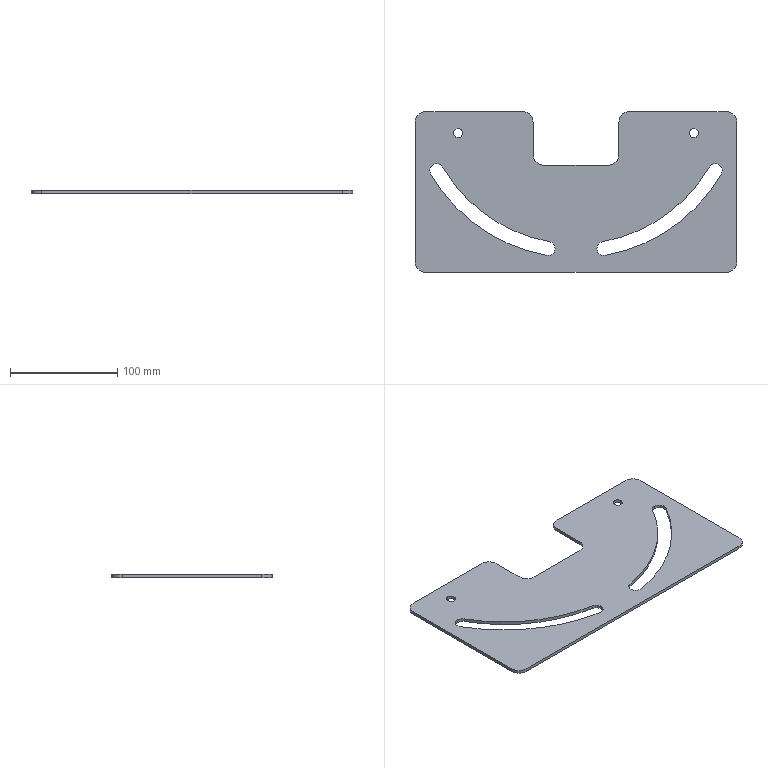Component | SolidWorks | KSD171005A-01-01-32-1 | 1 solid | 32 faces | box 300 x 150 x 3 mm | volume 111395 mm3 | cylinder 22 | plane 10 | commonest cylinder face diameters 20 x8 13 x6 8.5 x4 287 x2 313 x2
build123d program:
from build123d import *

# Parameters (mm, degrees)
SKETCH1_W                      = 150
SKETCH1_H                      = 300
BOSS_EXTRUDE1_DEPTH            = 3
CUT_EXTRUDE2_DEPTH             = 10
FILLET1_R                      = 10
SKETCH5_W                      = 100
SKETCH5_H                      = 80
CUT_EXTRUDE3_DEPTH             = 10
F_8_5_8_5_DIAMETER_HOLE1_D     = 8.5
F_8_5_8_5_DIAMETER_HOLE1_DEPTH = 11
F_8_5_8_5_DIAMETER_HOLE1_TIP   = 2.554
FILLET2_R                      = 10


with BuildPart() as part:
    # Sketch1 → Boss-Extrude1 (new body)
    with BuildSketch(Plane.XY):
        Rectangle(SKETCH1_W, SKETCH1_H)
    extrude(amount=BOSS_EXTRUDE1_DEPTH)

    # Sketch4 → Cut-Extrude2 (cut)
    with BuildSketch(Plane.XY.offset(3)):
        with BuildLine():
            ThreePointArc((16.75, 135.533), (-33.197, 89.765), (-59.122, 27.176))
            ThreePointArc((-59.122, 27.176), (-53.85, 19.646), (-46.32, 24.919))
            ThreePointArc((-46.32, 24.919), (-22.548, 82.308), (23.25, 124.275))
            ThreePointArc((23.25, 124.275), (25.629, 133.154), (16.75, 135.533))
        make_face()
        with BuildLine():
            ThreePointArc((16.75, -135.533), (-33.197, -89.765), (-59.122, -27.176))
            ThreePointArc((-59.122, -27.176), (-53.85, -19.646), (-46.32, -24.919))
            ThreePointArc((-46.32, -24.919), (-22.548, -82.308), (23.25, -124.275))
            ThreePointArc((23.25, -124.275), (25.629, -133.154), (16.75, -135.533))
        make_face()
    extrude(amount=-CUT_EXTRUDE2_DEPTH, mode=Mode.SUBTRACT)

    # Fillet1
    fillet1_edges = [part.edges().sort_by_distance(p)[0] for p in [
        (75, -150, 1.5),
        (-75, -150, 1.5),
        (-75, 150, 1.5),
        (75, 150, 1.5),
    ]]
    fillet(fillet1_edges, radius=FILLET1_R)

    # Sketch5 → Cut-Extrude3 (cut)
    with BuildSketch(Plane.XY.offset(3)):
        with Locations((75, 0)):
            Rectangle(SKETCH5_W, SKETCH5_H)
    extrude(amount=-CUT_EXTRUDE3_DEPTH, mode=Mode.SUBTRACT)

    # 8.5 _8.5_ Diameter Hole1
    with Locations(Plane.XY.offset(3)):
        with Locations((55, 110), (55, -110)):
            Hole(F_8_5_8_5_DIAMETER_HOLE1_D / 2, depth=F_8_5_8_5_DIAMETER_HOLE1_DEPTH)
            with Locations((0, 0, -(F_8_5_8_5_DIAMETER_HOLE1_DEPTH + F_8_5_8_5_DIAMETER_HOLE1_TIP / 2))):  # 118° drill point
                Cone(0, F_8_5_8_5_DIAMETER_HOLE1_D / 2, F_8_5_8_5_DIAMETER_HOLE1_TIP, mode=Mode.SUBTRACT)

    # Fillet2
    fillet2_edges = [part.edges().sort_by_distance(p)[0] for p in [
        (75, 40, 1.5),
        (75, -40, 1.5),
        (25, -40, 1.5),
        (25, 40, 1.5),
    ]]
    fillet(fillet2_edges, radius=FILLET2_R)


solid = part.part

# Placed as in the assembly
solid = solid.moved(Location((-7.111, -79.27, 348), (0, 0, 90)))
STEP:
#1=CARTESIAN_POINT('',(-4.611,-1.123,13.701));
#2=VERTEX_POINT('',#1);
#3=CARTESIAN_POINT('',(-4.611,-0.7882,13.701));
#4=VERTEX_POINT('',#3);
#5=CARTESIAN_POINT('',(-4.611,-0.9555,13.701));
#6=DIRECTION('',(-0.,-0.,1.));
#7=DIRECTION('',(0.,1.,0.));
#8=AXIS2_PLACEMENT_3D('',#5,#6,#7);
#9=CIRCLE('',#8,0.1673);
#10=EDGE_CURVE('',#2,#4,#9,.T.);
#11=ORIENTED_EDGE('',*,*,#10,.F.);
#12=CARTESIAN_POINT('',(-4.611,-1.123,13.819));
#13=VERTEX_POINT('',#12);
#14=CARTESIAN_POINT('',(-4.611,-1.123,13.819));
#15=DIRECTION('',(-0.,-0.,1.));
#16=VECTOR('',#15,39.37);
#17=LINE('',#14,#16);
#18=EDGE_CURVE('',#2,#13,#17,.T.);
#19=ORIENTED_EDGE('',*,*,#18,.T.);
#20=CARTESIAN_POINT('',(-4.611,-0.7882,13.819));
#21=VERTEX_POINT('',#20);
#22=CARTESIAN_POINT('',(-4.611,-0.9555,13.819));
#23=DIRECTION('',(-0.,-0.,1.));
#24=DIRECTION('',(0.,1.,0.));
#25=AXIS2_PLACEMENT_3D('',#22,#23,#24);
#26=CIRCLE('',#25,0.1673);
#27=EDGE_CURVE('',#13,#21,#26,.T.);
#28=ORIENTED_EDGE('',*,*,#27,.T.);
#29=CARTESIAN_POINT('',(-4.611,-0.7882,13.819));
#30=DIRECTION('',(-0.,-0.,1.));
#31=VECTOR('',#30,39.37);
#32=LINE('',#29,#31);
#33=EDGE_CURVE('',#4,#21,#32,.T.);
#34=ORIENTED_EDGE('',*,*,#33,.F.);
#35=EDGE_LOOP('',(#11,#19,#28,#34));
#36=FACE_OUTER_BOUND('',#35,.T.);
#37=CARTESIAN_POINT('',(-4.611,-0.9555,13.819));
#38=DIRECTION('',(-0.,-0.,1.));
#39=DIRECTION('',(0.,1.,0.));
#40=AXIS2_PLACEMENT_3D('',#37,#38,#39);
#41=CYLINDRICAL_SURFACE('',#40,0.1673);
#42=ADVANCED_FACE('',(#36),#41,.F.);
#43=CARTESIAN_POINT('',(4.051,-1.123,13.701));
#44=VERTEX_POINT('',#43);
#45=CARTESIAN_POINT('',(4.051,-0.7882,13.701));
#46=VERTEX_POINT('',#45);
#47=CARTESIAN_POINT('',(4.051,-0.9555,13.701));
#48=DIRECTION('',(-0.,-0.,1.));
#49=DIRECTION('',(0.,1.,0.));
#50=AXIS2_PLACEMENT_3D('',#47,#48,#49);
#51=CIRCLE('',#50,0.1673);
#52=EDGE_CURVE('',#44,#46,#51,.T.);
#53=ORIENTED_EDGE('',*,*,#52,.F.);
#54=CARTESIAN_POINT('',(4.051,-1.123,13.819));
#55=VERTEX_POINT('',#54);
#56=CARTESIAN_POINT('',(4.051,-1.123,13.819));
#57=DIRECTION('',(-0.,-0.,1.));
#58=VECTOR('',#57,39.37);
#59=LINE('',#56,#58);
#60=EDGE_CURVE('',#44,#55,#59,.T.);
#61=ORIENTED_EDGE('',*,*,#60,.T.);
#62=CARTESIAN_POINT('',(4.051,-0.7882,13.819));
#63=VERTEX_POINT('',#62);
#64=CARTESIAN_POINT('',(4.051,-0.9555,13.819));
#65=DIRECTION('',(-0.,-0.,1.));
#66=DIRECTION('',(0.,1.,0.));
#67=AXIS2_PLACEMENT_3D('',#64,#65,#66);
#68=CIRCLE('',#67,0.1673);
#69=EDGE_CURVE('',#55,#63,#68,.T.);
#70=ORIENTED_EDGE('',*,*,#69,.T.);
#71=CARTESIAN_POINT('',(4.051,-0.7882,13.819));
#72=DIRECTION('',(-0.,-0.,1.));
#73=VECTOR('',#72,39.37);
#74=LINE('',#71,#73);
#75=EDGE_CURVE('',#46,#63,#74,.T.);
#76=ORIENTED_EDGE('',*,*,#75,.F.);
#77=EDGE_LOOP('',(#53,#61,#70,#76));
#78=FACE_OUTER_BOUND('',#77,.T.);
#79=CARTESIAN_POINT('',(4.051,-0.9555,13.819));
#80=DIRECTION('',(-0.,-0.,1.));
#81=DIRECTION('',(0.,1.,0.));
#82=AXIS2_PLACEMENT_3D('',#79,#80,#81);
#83=CYLINDRICAL_SURFACE('',#82,0.1673);
#84=ADVANCED_FACE('',(#78),#83,.F.);
#85=CARTESIAN_POINT('',(4.834,-2.078,13.701));
#86=VERTEX_POINT('',#85);
#87=CARTESIAN_POINT('',(4.613,-2.206,13.701));
#88=VERTEX_POINT('',#87);
#89=CARTESIAN_POINT('',(4.834,-2.333,13.701));
#90=DIRECTION('',(-0.,-0.,1.));
#91=DIRECTION('',(0.,1.,0.));
#92=AXIS2_PLACEMENT_3D('',#89,#90,#91);
#93=CIRCLE('',#92,0.2559);
#94=EDGE_CURVE('',#86,#88,#93,.T.);
#95=ORIENTED_EDGE('',*,*,#94,.F.);
#96=CARTESIAN_POINT('',(4.834,-2.078,13.819));
#97=VERTEX_POINT('',#96);
#98=CARTESIAN_POINT('',(4.834,-2.078,13.425));
#99=DIRECTION('',(-0.,-0.,1.));
#100=VECTOR('',#99,39.37);
#101=LINE('',#98,#100);
#102=EDGE_CURVE('',#86,#97,#101,.T.);
#103=ORIENTED_EDGE('',*,*,#102,.T.);
#104=CARTESIAN_POINT('',(4.613,-2.206,13.819));
#105=VERTEX_POINT('',#104);
#106=CARTESIAN_POINT('',(4.834,-2.333,13.819));
#107=DIRECTION('',(-0.,-0.,1.));
#108=DIRECTION('',(0.,-1.,0.));
#109=AXIS2_PLACEMENT_3D('',#106,#107,#108);
#110=CIRCLE('',#109,0.2559);
#111=EDGE_CURVE('',#97,#105,#110,.T.);
#112=ORIENTED_EDGE('',*,*,#111,.T.);
#113=CARTESIAN_POINT('',(4.613,-2.206,13.425));
#114=DIRECTION('',(-0.,-0.,1.));
#115=VECTOR('',#114,39.37);
#116=LINE('',#113,#115);
#117=EDGE_CURVE('',#88,#105,#116,.T.);
#118=ORIENTED_EDGE('',*,*,#117,.F.);
#119=EDGE_LOOP('',(#95,#103,#112,#118));
#120=FACE_OUTER_BOUND('',#119,.T.);
#121=CARTESIAN_POINT('',(4.834,-2.333,13.425));
#122=DIRECTION('',(-0.,-0.,1.));
#123=DIRECTION('',(0.,1.,0.));
#124=AXIS2_PLACEMENT_3D('',#121,#122,#123);
#125=CYLINDRICAL_SURFACE('',#124,0.2559);
#126=ADVANCED_FACE('',(#120),#125,.F.);
#127=CARTESIAN_POINT('',(-5.394,-2.078,13.701));
#128=VERTEX_POINT('',#127);
#129=CARTESIAN_POINT('',(-5.616,-2.461,13.701));
#130=VERTEX_POINT('',#129);
#131=CARTESIAN_POINT('',(-5.394,-2.333,13.701));
#132=DIRECTION('',(-0.,-0.,1.));
#133=DIRECTION('',(0.,1.,0.));
#134=AXIS2_PLACEMENT_3D('',#131,#132,#133);
#135=CIRCLE('',#134,0.2559);
#136=EDGE_CURVE('',#128,#130,#135,.T.);
#137=ORIENTED_EDGE('',*,*,#136,.F.);
#138=CARTESIAN_POINT('',(-5.394,-2.078,13.819));
#139=VERTEX_POINT('',#138);
#140=CARTESIAN_POINT('',(-5.394,-2.078,13.425));
#141=DIRECTION('',(-0.,-0.,1.));
#142=VECTOR('',#141,39.37);
#143=LINE('',#140,#142);
#144=EDGE_CURVE('',#128,#139,#143,.T.);
#145=ORIENTED_EDGE('',*,*,#144,.T.);
#146=CARTESIAN_POINT('',(-5.616,-2.461,13.819));
#147=VERTEX_POINT('',#146);
#148=CARTESIAN_POINT('',(-5.394,-2.333,13.819));
#149=DIRECTION('',(-0.,-0.,1.));
#150=DIRECTION('',(0.,1.,0.));
#151=AXIS2_PLACEMENT_3D('',#148,#149,#150);
#152=CIRCLE('',#151,0.2559);
#153=EDGE_CURVE('',#139,#147,#152,.T.);
#154=ORIENTED_EDGE('',*,*,#153,.T.);
#155=CARTESIAN_POINT('',(-5.616,-2.461,13.425));
#156=DIRECTION('',(-0.,-0.,1.));
#157=VECTOR('',#156,39.37);
#158=LINE('',#155,#157);
#159=EDGE_CURVE('',#130,#147,#158,.T.);
#160=ORIENTED_EDGE('',*,*,#159,.F.);
#161=EDGE_LOOP('',(#137,#145,#154,#160));
#162=FACE_OUTER_BOUND('',#161,.T.);
#163=CARTESIAN_POINT('',(-5.394,-2.333,13.425));
#164=DIRECTION('',(-0.,-0.,1.));
#165=DIRECTION('',(0.,1.,0.));
#166=AXIS2_PLACEMENT_3D('',#163,#164,#165);
#167=CYLINDRICAL_SURFACE('',#166,0.2559);
#168=ADVANCED_FACE('',(#162),#167,.F.);
#169=CARTESIAN_POINT('',(5.232,-0.1681,13.701));
#170=VERTEX_POINT('',#169);
#171=CARTESIAN_POINT('',(1.689,-0.1681,13.701));
#172=VERTEX_POINT('',#171);
#173=CARTESIAN_POINT('',(-6.185,-0.1681,13.701));
#174=DIRECTION('',(-1.,0.,-0.));
#175=VECTOR('',#174,39.37);
#176=LINE('',#173,#175);
#177=EDGE_CURVE('',#170,#172,#176,.T.);
#178=ORIENTED_EDGE('',*,*,#177,.T.);
#179=CARTESIAN_POINT('',(1.689,-0.1681,13.819));
#180=VERTEX_POINT('',#179);
#181=CARTESIAN_POINT('',(1.689,-0.1681,13.819));
#182=DIRECTION('',(-0.,-0.,1.));
#183=VECTOR('',#182,39.37);
#184=LINE('',#181,#183);
#185=EDGE_CURVE('',#172,#180,#184,.T.);
#186=ORIENTED_EDGE('',*,*,#185,.T.);
#187=CARTESIAN_POINT('',(5.232,-0.1681,13.819));
#188=VERTEX_POINT('',#187);
#189=CARTESIAN_POINT('',(-6.185,-0.1681,13.819));
#190=DIRECTION('',(-1.,0.,-0.));
#191=VECTOR('',#190,39.37);
#192=LINE('',#189,#191);
#193=EDGE_CURVE('',#188,#180,#192,.T.);
#194=ORIENTED_EDGE('',*,*,#193,.F.);
#195=CARTESIAN_POINT('',(5.232,-0.1681,13.819));
#196=DIRECTION('',(0.,0.,-1.));
#197=VECTOR('',#196,39.37);
#198=LINE('',#195,#197);
#199=EDGE_CURVE('',#188,#170,#198,.T.);
#200=ORIENTED_EDGE('',*,*,#199,.T.);
#201=EDGE_LOOP('',(#178,#186,#194,#200));
#202=FACE_OUTER_BOUND('',#201,.T.);
#203=CARTESIAN_POINT('',(-6.185,-0.1681,13.819));
#204=DIRECTION('',(-0.,-1.,-0.));
#205=DIRECTION('',(1.,-0.,0.));
#206=AXIS2_PLACEMENT_3D('',#203,#204,#205);
#207=PLANE('',#206);
#208=ADVANCED_FACE('',(#202),#207,.F.);
#209=CARTESIAN_POINT('',(-4.611,-0.9555,13.819));
#210=DIRECTION('',(-0.,-0.,1.));
#211=DIRECTION('',(0.,1.,0.));
#212=AXIS2_PLACEMENT_3D('',#209,#210,#211);
#213=CIRCLE('',#212,0.1673);
#214=EDGE_CURVE('',#21,#13,#213,.T.);
#215=ORIENTED_EDGE('',*,*,#214,.F.);
#216=ORIENTED_EDGE('',*,*,#27,.F.);
#217=EDGE_LOOP('',(#215,#216));
#218=FACE_BOUND('',#217,.T.);
#219=CARTESIAN_POINT('',(4.051,-0.9555,13.819));
#220=DIRECTION('',(-0.,-0.,1.));
#221=DIRECTION('',(0.,1.,0.));
#222=AXIS2_PLACEMENT_3D('',#219,#220,#221);
#223=CIRCLE('',#222,0.1673);
#224=EDGE_CURVE('',#63,#55,#223,.T.);
#225=ORIENTED_EDGE('',*,*,#224,.F.);
#226=ORIENTED_EDGE('',*,*,#69,.F.);
#227=EDGE_LOOP('',(#225,#226));
#228=FACE_BOUND('',#227,.T.);
#229=ORIENTED_EDGE('',*,*,#193,.T.);
#230=CARTESIAN_POINT('',(1.295,-0.5618,13.819));
#231=VERTEX_POINT('',#230);
#232=CARTESIAN_POINT('',(1.689,-0.5618,13.819));
#233=DIRECTION('',(-0.,-0.,1.));
#234=DIRECTION('',(0.,1.,0.));
#235=AXIS2_PLACEMENT_3D('',#232,#233,#234);
#236=CIRCLE('',#235,0.3937);
#237=EDGE_CURVE('',#180,#231,#236,.T.);
#238=ORIENTED_EDGE('',*,*,#237,.T.);
#239=CARTESIAN_POINT('',(1.295,-1.743,13.819));
#240=VERTEX_POINT('',#239);
#241=CARTESIAN_POINT('',(1.295,-2.137,13.819));
#242=DIRECTION('',(0.,1.,0.));
#243=VECTOR('',#242,39.37);
#244=LINE('',#241,#243);
#245=EDGE_CURVE('',#240,#231,#244,.T.);
#246=ORIENTED_EDGE('',*,*,#245,.F.);
#247=CARTESIAN_POINT('',(0.9011,-2.137,13.819));
#248=VERTEX_POINT('',#247);
#249=CARTESIAN_POINT('',(0.9011,-1.743,13.819));
#250=DIRECTION('',(0.,0.,-1.));
#251=DIRECTION('',(0.,1.,0.));
#252=AXIS2_PLACEMENT_3D('',#249,#250,#251);
#253=CIRCLE('',#252,0.3937);
#254=EDGE_CURVE('',#240,#248,#253,.T.);
#255=ORIENTED_EDGE('',*,*,#254,.T.);
#256=CARTESIAN_POINT('',(-1.461,-2.137,13.819));
#257=VERTEX_POINT('',#256);
#258=CARTESIAN_POINT('',(-1.855,-2.137,13.819));
#259=DIRECTION('',(1.,-0.,0.));
#260=VECTOR('',#259,39.37);
#261=LINE('',#258,#260);
#262=EDGE_CURVE('',#257,#248,#261,.T.);
#263=ORIENTED_EDGE('',*,*,#262,.F.);
#264=CARTESIAN_POINT('',(-1.855,-1.743,13.819));
#265=VERTEX_POINT('',#264);
#266=CARTESIAN_POINT('',(-1.461,-1.743,13.819));
#267=DIRECTION('',(0.,0.,-1.));
#268=DIRECTION('',(0.,1.,0.));
#269=AXIS2_PLACEMENT_3D('',#266,#267,#268);
#270=CIRCLE('',#269,0.3937);
#271=EDGE_CURVE('',#257,#265,#270,.T.);
#272=ORIENTED_EDGE('',*,*,#271,.T.);
#273=CARTESIAN_POINT('',(-1.855,-0.5618,13.819));
#274=VERTEX_POINT('',#273);
#275=CARTESIAN_POINT('',(-1.855,-2.137,13.819));
#276=DIRECTION('',(-0.,-1.,-0.));
#277=VECTOR('',#276,39.37);
#278=LINE('',#275,#277);
#279=EDGE_CURVE('',#274,#265,#278,.T.);
#280=ORIENTED_EDGE('',*,*,#279,.F.);
#281=CARTESIAN_POINT('',(-2.248,-0.1681,13.819));
#282=VERTEX_POINT('',#281);
#283=CARTESIAN_POINT('',(-2.248,-0.5618,13.819));
#284=DIRECTION('',(-0.,-0.,1.));
#285=DIRECTION('',(0.,1.,0.));
#286=AXIS2_PLACEMENT_3D('',#283,#284,#285);
#287=CIRCLE('',#286,0.3937);
#288=EDGE_CURVE('',#274,#282,#287,.T.);
#289=ORIENTED_EDGE('',*,*,#288,.T.);
#290=CARTESIAN_POINT('',(-5.792,-0.1681,13.819));
#291=VERTEX_POINT('',#290);
#292=CARTESIAN_POINT('',(-6.185,-0.1681,13.819));
#293=DIRECTION('',(-1.,0.,-0.));
#294=VECTOR('',#293,39.37);
#295=LINE('',#292,#294);
#296=EDGE_CURVE('',#282,#291,#295,.T.);
#297=ORIENTED_EDGE('',*,*,#296,.T.);
#298=CARTESIAN_POINT('',(-6.185,-0.5618,13.819));
#299=VERTEX_POINT('',#298);
#300=CARTESIAN_POINT('',(-5.792,-0.5618,13.819));
#301=DIRECTION('',(-0.,-0.,1.));
#302=DIRECTION('',(0.,1.,0.));
#303=AXIS2_PLACEMENT_3D('',#300,#301,#302);
#304=CIRCLE('',#303,0.3937);
#305=EDGE_CURVE('',#291,#299,#304,.T.);
#306=ORIENTED_EDGE('',*,*,#305,.T.);
#307=CARTESIAN_POINT('',(-6.185,-5.68,13.819));
#308=VERTEX_POINT('',#307);
#309=CARTESIAN_POINT('',(-6.185,-6.074,13.819));
#310=DIRECTION('',(-0.,-1.,-0.));
#311=VECTOR('',#310,39.37);
#312=LINE('',#309,#311);
#313=EDGE_CURVE('',#299,#308,#312,.T.);
#314=ORIENTED_EDGE('',*,*,#313,.T.);
#315=CARTESIAN_POINT('',(-5.792,-6.074,13.819));
#316=VERTEX_POINT('',#315);
#317=CARTESIAN_POINT('',(-5.792,-5.68,13.819));
#318=DIRECTION('',(-0.,-0.,1.));
#319=DIRECTION('',(0.,1.,0.));
#320=AXIS2_PLACEMENT_3D('',#317,#318,#319);
#321=CIRCLE('',#320,0.3937);
#322=EDGE_CURVE('',#308,#316,#321,.T.);
#323=ORIENTED_EDGE('',*,*,#322,.T.);
#324=CARTESIAN_POINT('',(5.232,-6.074,13.819));
#325=VERTEX_POINT('',#324);
#326=CARTESIAN_POINT('',(-6.185,-6.074,13.819));
#327=DIRECTION('',(1.,-0.,0.));
#328=VECTOR('',#327,39.37);
#329=LINE('',#326,#328);
#330=EDGE_CURVE('',#316,#325,#329,.T.);
#331=ORIENTED_EDGE('',*,*,#330,.T.);
#332=CARTESIAN_POINT('',(5.626,-5.68,13.819));
#333=VERTEX_POINT('',#332);
#334=CARTESIAN_POINT('',(5.232,-5.68,13.819));
#335=DIRECTION('',(-0.,-0.,1.));
#336=DIRECTION('',(0.,1.,0.));
#337=AXIS2_PLACEMENT_3D('',#334,#335,#336);
#338=CIRCLE('',#337,0.3937);
#339=EDGE_CURVE('',#325,#333,#338,.T.);
#340=ORIENTED_EDGE('',*,*,#339,.T.);
#341=CARTESIAN_POINT('',(5.626,-0.5618,13.819));
#342=VERTEX_POINT('',#341);
#343=CARTESIAN_POINT('',(5.626,-6.074,13.819));
#344=DIRECTION('',(0.,1.,0.));
#345=VECTOR('',#344,39.37);
#346=LINE('',#343,#345);
#347=EDGE_CURVE('',#333,#342,#346,.T.);
#348=ORIENTED_EDGE('',*,*,#347,.T.);
#349=CARTESIAN_POINT('',(5.232,-0.5618,13.819));
#350=DIRECTION('',(-0.,-0.,1.));
#351=DIRECTION('',(0.,1.,0.));
#352=AXIS2_PLACEMENT_3D('',#349,#350,#351);
#353=CIRCLE('',#352,0.3937);
#354=EDGE_CURVE('',#342,#188,#353,.T.);
#355=ORIENTED_EDGE('',*,*,#354,.T.);
#356=EDGE_LOOP('',(#229,#238,#246,#255,#263,#272,#280,#289,#297,#306,#314,#323,#331,#340,#348,#355));
#357=FACE_OUTER_BOUND('',#356,.T.);
#358=CARTESIAN_POINT('',(-5.173,-2.206,13.819));
#359=VERTEX_POINT('',#358);
#360=CARTESIAN_POINT('',(-5.394,-2.333,13.819));
#361=DIRECTION('',(-0.,-0.,1.));
#362=DIRECTION('',(0.,1.,0.));
#363=AXIS2_PLACEMENT_3D('',#360,#361,#362);
#364=CIRCLE('',#363,0.2559);
#365=EDGE_CURVE('',#359,#139,#364,.T.);
#366=ORIENTED_EDGE('',*,*,#365,.F.);
#367=CARTESIAN_POINT('',(-1.261,-4.944,13.819));
#368=VERTEX_POINT('',#367);
#369=CARTESIAN_POINT('',(-0.28,0.6193,13.819));
#370=DIRECTION('',(0.,0.,-1.));
#371=DIRECTION('',(0.,1.,0.));
#372=AXIS2_PLACEMENT_3D('',#369,#370,#371);
#373=CIRCLE('',#372,5.65);
#374=EDGE_CURVE('',#368,#359,#373,.T.);
#375=ORIENTED_EDGE('',*,*,#374,.F.);
#376=CARTESIAN_POINT('',(-1.35,-5.449,13.819));
#377=VERTEX_POINT('',#376);
#378=CARTESIAN_POINT('',(-1.305,-5.197,13.819));
#379=DIRECTION('',(-0.,-0.,1.));
#380=DIRECTION('',(0.,1.,0.));
#381=AXIS2_PLACEMENT_3D('',#378,#379,#380);
#382=CIRCLE('',#381,0.2559);
#383=EDGE_CURVE('',#377,#368,#382,.T.);
#384=ORIENTED_EDGE('',*,*,#383,.F.);
#385=CARTESIAN_POINT('',(-0.28,0.6193,13.819));
#386=DIRECTION('',(-0.,-0.,1.));
#387=DIRECTION('',(0.,1.,0.));
#388=AXIS2_PLACEMENT_3D('',#385,#386,#387);
#389=CIRCLE('',#388,6.161);
#390=EDGE_CURVE('',#147,#377,#389,.T.);
#391=ORIENTED_EDGE('',*,*,#390,.F.);
#392=ORIENTED_EDGE('',*,*,#153,.F.);
#393=EDGE_LOOP('',(#366,#375,#384,#391,#392));
#394=FACE_BOUND('',#393,.T.);
#395=CARTESIAN_POINT('',(5.056,-2.461,13.819));
#396=VERTEX_POINT('',#395);
#397=CARTESIAN_POINT('',(4.834,-2.333,13.819));
#398=DIRECTION('',(-0.,-0.,1.));
#399=DIRECTION('',(0.,-1.,0.));
#400=AXIS2_PLACEMENT_3D('',#397,#398,#399);
#401=CIRCLE('',#400,0.2559);
#402=EDGE_CURVE('',#396,#97,#401,.T.);
#403=ORIENTED_EDGE('',*,*,#402,.F.);
#404=CARTESIAN_POINT('',(0.7899,-5.449,13.819));
#405=VERTEX_POINT('',#404);
#406=CARTESIAN_POINT('',(-0.28,0.6193,13.819));
#407=DIRECTION('',(-0.,-0.,1.));
#408=DIRECTION('',(-0.,-1.,0.));
#409=AXIS2_PLACEMENT_3D('',#406,#407,#408);
#410=CIRCLE('',#409,6.161);
#411=EDGE_CURVE('',#405,#396,#410,.T.);
#412=ORIENTED_EDGE('',*,*,#411,.F.);
#413=CARTESIAN_POINT('',(0.7011,-4.944,13.819));
#414=VERTEX_POINT('',#413);
#415=CARTESIAN_POINT('',(0.7455,-5.197,13.819));
#416=DIRECTION('',(-0.,-0.,1.));
#417=DIRECTION('',(0.,-1.,0.));
#418=AXIS2_PLACEMENT_3D('',#415,#416,#417);
#419=CIRCLE('',#418,0.2559);
#420=EDGE_CURVE('',#414,#405,#419,.T.);
#421=ORIENTED_EDGE('',*,*,#420,.F.);
#422=CARTESIAN_POINT('',(-0.28,0.6193,13.819));
#423=DIRECTION('',(0.,0.,-1.));
#424=DIRECTION('',(-0.,-1.,0.));
#425=AXIS2_PLACEMENT_3D('',#422,#423,#424);
#426=CIRCLE('',#425,5.65);
#427=EDGE_CURVE('',#105,#414,#426,.T.);
#428=ORIENTED_EDGE('',*,*,#427,.F.);
#429=ORIENTED_EDGE('',*,*,#111,.F.);
#430=EDGE_LOOP('',(#403,#412,#421,#428,#429));
#431=FACE_BOUND('',#430,.T.);
#432=CARTESIAN_POINT('',(-0.28,-3.121,13.819));
#433=DIRECTION('',(-0.,-0.,1.));
#434=DIRECTION('',(0.,1.,0.));
#435=AXIS2_PLACEMENT_3D('',#432,#433,#434);
#436=PLANE('',#435);
#437=ADVANCED_FACE('',(#218,#228,#357,#394,#431),#436,.T.);
#438=CARTESIAN_POINT('',(-4.611,-0.9555,13.701));
#439=DIRECTION('',(-0.,-0.,1.));
#440=DIRECTION('',(0.,1.,0.));
#441=AXIS2_PLACEMENT_3D('',#438,#439,#440);
#442=CIRCLE('',#441,0.1673);
#443=EDGE_CURVE('',#4,#2,#442,.T.);
#444=ORIENTED_EDGE('',*,*,#443,.T.);
#445=ORIENTED_EDGE('',*,*,#10,.T.);
#446=EDGE_LOOP('',(#444,#445));
#447=FACE_BOUND('',#446,.T.);
#448=CARTESIAN_POINT('',(4.051,-0.9555,13.701));
#449=DIRECTION('',(-0.,-0.,1.));
#450=DIRECTION('',(0.,1.,0.));
#451=AXIS2_PLACEMENT_3D('',#448,#449,#450);
#452=CIRCLE('',#451,0.1673);
#453=EDGE_CURVE('',#46,#44,#452,.T.);
#454=ORIENTED_EDGE('',*,*,#453,.T.);
#455=ORIENTED_EDGE('',*,*,#52,.T.);
#456=EDGE_LOOP('',(#454,#455));
#457=FACE_BOUND('',#456,.T.);
#458=CARTESIAN_POINT('',(-1.261,-4.944,13.701));
#459=VERTEX_POINT('',#458);
#460=CARTESIAN_POINT('',(-5.173,-2.206,13.701));
#461=VERTEX_POINT('',#460);
#462=CARTESIAN_POINT('',(-0.28,0.6193,13.701));
#463=DIRECTION('',(0.,0.,-1.));
#464=DIRECTION('',(0.,1.,0.));
#465=AXIS2_PLACEMENT_3D('',#462,#463,#464);
#466=CIRCLE('',#465,5.65);
#467=EDGE_CURVE('',#459,#461,#466,.T.);
#468=ORIENTED_EDGE('',*,*,#467,.T.);
#469=CARTESIAN_POINT('',(-5.394,-2.333,13.701));
#470=DIRECTION('',(-0.,-0.,1.));
#471=DIRECTION('',(0.,1.,0.));
#472=AXIS2_PLACEMENT_3D('',#469,#470,#471);
#473=CIRCLE('',#472,0.2559);
#474=EDGE_CURVE('',#461,#128,#473,.T.);
#475=ORIENTED_EDGE('',*,*,#474,.T.);
#476=ORIENTED_EDGE('',*,*,#136,.T.);
#477=CARTESIAN_POINT('',(-1.35,-5.449,13.701));
#478=VERTEX_POINT('',#477);
#479=CARTESIAN_POINT('',(-0.28,0.6193,13.701));
#480=DIRECTION('',(-0.,-0.,1.));
#481=DIRECTION('',(0.,1.,0.));
#482=AXIS2_PLACEMENT_3D('',#479,#480,#481);
#483=CIRCLE('',#482,6.161);
#484=EDGE_CURVE('',#130,#478,#483,.T.);
#485=ORIENTED_EDGE('',*,*,#484,.T.);
#486=CARTESIAN_POINT('',(-1.305,-5.197,13.701));
#487=DIRECTION('',(-0.,-0.,1.));
#488=DIRECTION('',(0.,1.,0.));
#489=AXIS2_PLACEMENT_3D('',#486,#487,#488);
#490=CIRCLE('',#489,0.2559);
#491=EDGE_CURVE('',#478,#459,#490,.T.);
#492=ORIENTED_EDGE('',*,*,#491,.T.);
#493=EDGE_LOOP('',(#468,#475,#476,#485,#492));
#494=FACE_BOUND('',#493,.T.);
#495=CARTESIAN_POINT('',(1.295,-1.743,13.701));
#496=VERTEX_POINT('',#495);
#497=CARTESIAN_POINT('',(1.295,-0.5618,13.701));
#498=VERTEX_POINT('',#497);
#499=CARTESIAN_POINT('',(1.295,-3.121,13.701));
#500=DIRECTION('',(0.,1.,0.));
#501=VECTOR('',#500,39.37);
#502=LINE('',#499,#501);
#503=EDGE_CURVE('',#496,#498,#502,.T.);
#504=ORIENTED_EDGE('',*,*,#503,.T.);
#505=CARTESIAN_POINT('',(1.689,-0.5618,13.701));
#506=DIRECTION('',(0.,0.,-1.));
#507=DIRECTION('',(-0.,1.,0.));
#508=AXIS2_PLACEMENT_3D('',#505,#506,#507);
#509=CIRCLE('',#508,0.3937);
#510=EDGE_CURVE('',#498,#172,#509,.T.);
#511=ORIENTED_EDGE('',*,*,#510,.T.);
#512=ORIENTED_EDGE('',*,*,#177,.F.);
#513=CARTESIAN_POINT('',(5.626,-0.5618,13.701));
#514=VERTEX_POINT('',#513);
#515=CARTESIAN_POINT('',(5.232,-0.5618,13.701));
#516=DIRECTION('',(0.,0.,-1.));
#517=DIRECTION('',(0.,1.,0.));
#518=AXIS2_PLACEMENT_3D('',#515,#516,#517);
#519=CIRCLE('',#518,0.3937);
#520=EDGE_CURVE('',#170,#514,#519,.T.);
#521=ORIENTED_EDGE('',*,*,#520,.T.);
#522=CARTESIAN_POINT('',(5.626,-5.68,13.701));
#523=VERTEX_POINT('',#522);
#524=CARTESIAN_POINT('',(5.626,-6.074,13.701));
#525=DIRECTION('',(0.,1.,0.));
#526=VECTOR('',#525,39.37);
#527=LINE('',#524,#526);
#528=EDGE_CURVE('',#523,#514,#527,.T.);
#529=ORIENTED_EDGE('',*,*,#528,.F.);
#530=CARTESIAN_POINT('',(5.232,-6.074,13.701));
#531=VERTEX_POINT('',#530);
#532=CARTESIAN_POINT('',(5.232,-5.68,13.701));
#533=DIRECTION('',(0.,0.,-1.));
#534=DIRECTION('',(0.,1.,0.));
#535=AXIS2_PLACEMENT_3D('',#532,#533,#534);
#536=CIRCLE('',#535,0.3937);
#537=EDGE_CURVE('',#523,#531,#536,.T.);
#538=ORIENTED_EDGE('',*,*,#537,.T.);
#539=CARTESIAN_POINT('',(-5.792,-6.074,13.701));
#540=VERTEX_POINT('',#539);
#541=CARTESIAN_POINT('',(-6.185,-6.074,13.701));
#542=DIRECTION('',(1.,-0.,0.));
#543=VECTOR('',#542,39.37);
#544=LINE('',#541,#543);
#545=EDGE_CURVE('',#540,#531,#544,.T.);
#546=ORIENTED_EDGE('',*,*,#545,.F.);
#547=CARTESIAN_POINT('',(-6.185,-5.68,13.701));
#548=VERTEX_POINT('',#547);
#549=CARTESIAN_POINT('',(-5.792,-5.68,13.701));
#550=DIRECTION('',(0.,0.,-1.));
#551=DIRECTION('',(0.,1.,0.));
#552=AXIS2_PLACEMENT_3D('',#549,#550,#551);
#553=CIRCLE('',#552,0.3937);
#554=EDGE_CURVE('',#540,#548,#553,.T.);
#555=ORIENTED_EDGE('',*,*,#554,.T.);
#556=CARTESIAN_POINT('',(-6.185,-0.5618,13.701));
#557=VERTEX_POINT('',#556);
#558=CARTESIAN_POINT('',(-6.185,-6.074,13.701));
#559=DIRECTION('',(-0.,-1.,-0.));
#560=VECTOR('',#559,39.37);
#561=LINE('',#558,#560);
#562=EDGE_CURVE('',#557,#548,#561,.T.);
#563=ORIENTED_EDGE('',*,*,#562,.F.);
#564=CARTESIAN_POINT('',(-5.792,-0.1681,13.701));
#565=VERTEX_POINT('',#564);
#566=CARTESIAN_POINT('',(-5.792,-0.5618,13.701));
#567=DIRECTION('',(0.,0.,-1.));
#568=DIRECTION('',(0.,1.,0.));
#569=AXIS2_PLACEMENT_3D('',#566,#567,#568);
#570=CIRCLE('',#569,0.3937);
#571=EDGE_CURVE('',#557,#565,#570,.T.);
#572=ORIENTED_EDGE('',*,*,#571,.T.);
#573=CARTESIAN_POINT('',(-2.248,-0.1681,13.701));
#574=VERTEX_POINT('',#573);
#575=CARTESIAN_POINT('',(-6.185,-0.1681,13.701));
#576=DIRECTION('',(-1.,0.,-0.));
#577=VECTOR('',#576,39.37);
#578=LINE('',#575,#577);
#579=EDGE_CURVE('',#574,#565,#578,.T.);
#580=ORIENTED_EDGE('',*,*,#579,.F.);
#581=CARTESIAN_POINT('',(-1.855,-0.5618,13.701));
#582=VERTEX_POINT('',#581);
#583=CARTESIAN_POINT('',(-2.248,-0.5618,13.701));
#584=DIRECTION('',(0.,0.,-1.));
#585=DIRECTION('',(0.,1.,0.));
#586=AXIS2_PLACEMENT_3D('',#583,#584,#585);
#587=CIRCLE('',#586,0.3937);
#588=EDGE_CURVE('',#574,#582,#587,.T.);
#589=ORIENTED_EDGE('',*,*,#588,.T.);
#590=CARTESIAN_POINT('',(-1.855,-1.743,13.701));
#591=VERTEX_POINT('',#590);
#592=CARTESIAN_POINT('',(-1.855,-3.121,13.701));
#593=DIRECTION('',(-0.,-1.,-0.));
#594=VECTOR('',#593,39.37);
#595=LINE('',#592,#594);
#596=EDGE_CURVE('',#582,#591,#595,.T.);
#597=ORIENTED_EDGE('',*,*,#596,.T.);
#598=CARTESIAN_POINT('',(-1.461,-2.137,13.701));
#599=VERTEX_POINT('',#598);
#600=CARTESIAN_POINT('',(-1.461,-1.743,13.701));
#601=DIRECTION('',(-0.,-0.,1.));
#602=DIRECTION('',(0.,1.,0.));
#603=AXIS2_PLACEMENT_3D('',#600,#601,#602);
#604=CIRCLE('',#603,0.3937);
#605=EDGE_CURVE('',#591,#599,#604,.T.);
#606=ORIENTED_EDGE('',*,*,#605,.T.);
#607=CARTESIAN_POINT('',(0.9011,-2.137,13.701));
#608=VERTEX_POINT('',#607);
#609=CARTESIAN_POINT('',(-0.28,-2.137,13.701));
#610=DIRECTION('',(1.,-0.,0.));
#611=VECTOR('',#610,39.37);
#612=LINE('',#609,#611);
#613=EDGE_CURVE('',#599,#608,#612,.T.);
#614=ORIENTED_EDGE('',*,*,#613,.T.);
#615=CARTESIAN_POINT('',(0.9011,-1.743,13.701));
#616=DIRECTION('',(-0.,-0.,1.));
#617=DIRECTION('',(0.,1.,0.));
#618=AXIS2_PLACEMENT_3D('',#615,#616,#617);
#619=CIRCLE('',#618,0.3937);
#620=EDGE_CURVE('',#608,#496,#619,.T.);
#621=ORIENTED_EDGE('',*,*,#620,.T.);
#622=EDGE_LOOP('',(#504,#511,#512,#521,#529,#538,#546,#555,#563,#572,#580,#589,#597,#606,#614,#621));
#623=FACE_OUTER_BOUND('',#622,.T.);
#624=CARTESIAN_POINT('',(0.7899,-5.449,13.701));
#625=VERTEX_POINT('',#624);
#626=CARTESIAN_POINT('',(5.056,-2.461,13.701));
#627=VERTEX_POINT('',#626);
#628=CARTESIAN_POINT('',(-0.28,0.6193,13.701));
#629=DIRECTION('',(-0.,-0.,1.));
#630=DIRECTION('',(0.,1.,0.));
#631=AXIS2_PLACEMENT_3D('',#628,#629,#630);
#632=CIRCLE('',#631,6.161);
#633=EDGE_CURVE('',#625,#627,#632,.T.);
#634=ORIENTED_EDGE('',*,*,#633,.T.);
#635=CARTESIAN_POINT('',(4.834,-2.333,13.701));
#636=DIRECTION('',(-0.,-0.,1.));
#637=DIRECTION('',(0.,1.,0.));
#638=AXIS2_PLACEMENT_3D('',#635,#636,#637);
#639=CIRCLE('',#638,0.2559);
#640=EDGE_CURVE('',#627,#86,#639,.T.);
#641=ORIENTED_EDGE('',*,*,#640,.T.);
#642=ORIENTED_EDGE('',*,*,#94,.T.);
#643=CARTESIAN_POINT('',(0.7011,-4.944,13.701));
#644=VERTEX_POINT('',#643);
#645=CARTESIAN_POINT('',(-0.28,0.6193,13.701));
#646=DIRECTION('',(0.,0.,-1.));
#647=DIRECTION('',(0.,1.,0.));
#648=AXIS2_PLACEMENT_3D('',#645,#646,#647);
#649=CIRCLE('',#648,5.65);
#650=EDGE_CURVE('',#88,#644,#649,.T.);
#651=ORIENTED_EDGE('',*,*,#650,.T.);
#652=CARTESIAN_POINT('',(0.7455,-5.197,13.701));
#653=DIRECTION('',(-0.,-0.,1.));
#654=DIRECTION('',(0.,1.,0.));
#655=AXIS2_PLACEMENT_3D('',#652,#653,#654);
#656=CIRCLE('',#655,0.2559);
#657=EDGE_CURVE('',#644,#625,#656,.T.);
#658=ORIENTED_EDGE('',*,*,#657,.T.);
#659=EDGE_LOOP('',(#634,#641,#642,#651,#658));
#660=FACE_BOUND('',#659,.T.);
#661=CARTESIAN_POINT('',(-0.28,-3.121,13.701));
#662=DIRECTION('',(-0.,-0.,1.));
#663=DIRECTION('',(0.,1.,0.));
#664=AXIS2_PLACEMENT_3D('',#661,#662,#663);
#665=PLANE('',#664);
#666=ADVANCED_FACE('',(#447,#457,#494,#623,#660),#665,.F.);
#667=ORIENTED_EDGE('',*,*,#296,.F.);
#668=CARTESIAN_POINT('',(-2.248,-0.1681,13.819));
#669=DIRECTION('',(0.,0.,-1.));
#670=VECTOR('',#669,39.37);
#671=LINE('',#668,#670);
#672=EDGE_CURVE('',#282,#574,#671,.T.);
#673=ORIENTED_EDGE('',*,*,#672,.T.);
#674=ORIENTED_EDGE('',*,*,#579,.T.);
#675=CARTESIAN_POINT('',(-5.792,-0.1681,13.819));
#676=DIRECTION('',(-0.,-0.,1.));
#677=VECTOR('',#676,39.37);
#678=LINE('',#675,#677);
#679=EDGE_CURVE('',#565,#291,#678,.T.);
#680=ORIENTED_EDGE('',*,*,#679,.T.);
#681=EDGE_LOOP('',(#667,#673,#674,#680));
#682=FACE_OUTER_BOUND('',#681,.T.);
#683=CARTESIAN_POINT('',(-6.185,-0.1681,13.819));
#684=DIRECTION('',(-0.,-1.,-0.));
#685=DIRECTION('',(1.,-0.,0.));
#686=AXIS2_PLACEMENT_3D('',#683,#684,#685);
#687=PLANE('',#686);
#688=ADVANCED_FACE('',(#682),#687,.F.);
#689=ORIENTED_EDGE('',*,*,#313,.F.);
#690=CARTESIAN_POINT('',(-6.185,-0.5618,13.819));
#691=DIRECTION('',(0.,0.,-1.));
#692=VECTOR('',#691,39.37);
#693=LINE('',#690,#692);
#694=EDGE_CURVE('',#299,#557,#693,.T.);
#695=ORIENTED_EDGE('',*,*,#694,.T.);
#696=ORIENTED_EDGE('',*,*,#562,.T.);
#697=CARTESIAN_POINT('',(-6.185,-5.68,13.819));
#698=DIRECTION('',(-0.,-0.,1.));
#699=VECTOR('',#698,39.37);
#700=LINE('',#697,#699);
#701=EDGE_CURVE('',#548,#308,#700,.T.);
#702=ORIENTED_EDGE('',*,*,#701,.T.);
#703=EDGE_LOOP('',(#689,#695,#696,#702));
#704=FACE_OUTER_BOUND('',#703,.T.);
#705=CARTESIAN_POINT('',(-6.185,-6.074,13.819));
#706=DIRECTION('',(1.,-0.,0.));
#707=DIRECTION('',(0.,0.,-1.));
#708=AXIS2_PLACEMENT_3D('',#705,#706,#707);
#709=PLANE('',#708);
#710=ADVANCED_FACE('',(#704),#709,.F.);
#711=ORIENTED_EDGE('',*,*,#545,.T.);
#712=CARTESIAN_POINT('',(5.232,-6.074,13.819));
#713=DIRECTION('',(-0.,-0.,1.));
#714=VECTOR('',#713,39.37);
#715=LINE('',#712,#714);
#716=EDGE_CURVE('',#531,#325,#715,.T.);
#717=ORIENTED_EDGE('',*,*,#716,.T.);
#718=ORIENTED_EDGE('',*,*,#330,.F.);
#719=CARTESIAN_POINT('',(-5.792,-6.074,13.819));
#720=DIRECTION('',(0.,0.,-1.));
#721=VECTOR('',#720,39.37);
#722=LINE('',#719,#721);
#723=EDGE_CURVE('',#316,#540,#722,.T.);
#724=ORIENTED_EDGE('',*,*,#723,.T.);
#725=EDGE_LOOP('',(#711,#717,#718,#724));
#726=FACE_OUTER_BOUND('',#725,.T.);
#727=CARTESIAN_POINT('',(-6.185,-6.074,13.819));
#728=DIRECTION('',(0.,1.,0.));
#729=DIRECTION('',(-1.,0.,-0.));
#730=AXIS2_PLACEMENT_3D('',#727,#728,#729);
#731=PLANE('',#730);
#732=ADVANCED_FACE('',(#726),#731,.F.);
#733=ORIENTED_EDGE('',*,*,#347,.F.);
#734=CARTESIAN_POINT('',(5.626,-5.68,13.819));
#735=DIRECTION('',(0.,0.,-1.));
#736=VECTOR('',#735,39.37);
#737=LINE('',#734,#736);
#738=EDGE_CURVE('',#333,#523,#737,.T.);
#739=ORIENTED_EDGE('',*,*,#738,.T.);
#740=ORIENTED_EDGE('',*,*,#528,.T.);
#741=CARTESIAN_POINT('',(5.626,-0.5618,13.819));
#742=DIRECTION('',(-0.,-0.,1.));
#743=VECTOR('',#742,39.37);
#744=LINE('',#741,#743);
#745=EDGE_CURVE('',#514,#342,#744,.T.);
#746=ORIENTED_EDGE('',*,*,#745,.T.);
#747=EDGE_LOOP('',(#733,#739,#740,#746));
#748=FACE_OUTER_BOUND('',#747,.T.);
#749=CARTESIAN_POINT('',(5.626,-6.074,13.819));
#750=DIRECTION('',(-1.,0.,-0.));
#751=DIRECTION('',(-0.,-0.,1.));
#752=AXIS2_PLACEMENT_3D('',#749,#750,#751);
#753=PLANE('',#752);
#754=ADVANCED_FACE('',(#748),#753,.F.);
#755=ORIENTED_EDGE('',*,*,#144,.F.);
#756=ORIENTED_EDGE('',*,*,#474,.F.);
#757=CARTESIAN_POINT('',(-5.173,-2.206,13.425));
#758=DIRECTION('',(-0.,-0.,1.));
#759=VECTOR('',#758,39.37);
#760=LINE('',#757,#759);
#761=EDGE_CURVE('',#461,#359,#760,.T.);
#762=ORIENTED_EDGE('',*,*,#761,.T.);
#763=ORIENTED_EDGE('',*,*,#365,.T.);
#764=EDGE_LOOP('',(#755,#756,#762,#763));
#765=FACE_OUTER_BOUND('',#764,.T.);
#766=CARTESIAN_POINT('',(-5.394,-2.333,13.425));
#767=DIRECTION('',(-0.,-0.,1.));
#768=DIRECTION('',(0.,1.,0.));
#769=AXIS2_PLACEMENT_3D('',#766,#767,#768);
#770=CYLINDRICAL_SURFACE('',#769,0.2559);
#771=ADVANCED_FACE('',(#765),#770,.F.);
#772=CARTESIAN_POINT('',(-1.261,-4.944,13.425));
#773=DIRECTION('',(-0.,-0.,1.));
#774=VECTOR('',#773,39.37);
#775=LINE('',#772,#774);
#776=EDGE_CURVE('',#459,#368,#775,.T.);
#777=ORIENTED_EDGE('',*,*,#776,.T.);
#778=ORIENTED_EDGE('',*,*,#374,.T.);
#779=ORIENTED_EDGE('',*,*,#761,.F.);
#780=ORIENTED_EDGE('',*,*,#467,.F.);
#781=EDGE_LOOP('',(#777,#778,#779,#780));
#782=FACE_OUTER_BOUND('',#781,.T.);
#783=CARTESIAN_POINT('',(-0.28,0.6193,13.425));
#784=DIRECTION('',(-0.,-0.,1.));
#785=DIRECTION('',(0.,1.,0.));
#786=AXIS2_PLACEMENT_3D('',#783,#784,#785);
#787=CYLINDRICAL_SURFACE('',#786,5.65);
#788=ADVANCED_FACE('',(#782),#787,.T.);
#789=CARTESIAN_POINT('',(-1.35,-5.449,13.425));
#790=DIRECTION('',(-0.,-0.,1.));
#791=VECTOR('',#790,39.37);
#792=LINE('',#789,#791);
#793=EDGE_CURVE('',#478,#377,#792,.T.);
#794=ORIENTED_EDGE('',*,*,#793,.T.);
#795=ORIENTED_EDGE('',*,*,#383,.T.);
#796=ORIENTED_EDGE('',*,*,#776,.F.);
#797=ORIENTED_EDGE('',*,*,#491,.F.);
#798=EDGE_LOOP('',(#794,#795,#796,#797));
#799=FACE_OUTER_BOUND('',#798,.T.);
#800=CARTESIAN_POINT('',(-1.305,-5.197,13.425));
#801=DIRECTION('',(-0.,-0.,1.));
#802=DIRECTION('',(0.,1.,0.));
#803=AXIS2_PLACEMENT_3D('',#800,#801,#802);
#804=CYLINDRICAL_SURFACE('',#803,0.2559);
#805=ADVANCED_FACE('',(#799),#804,.F.);
#806=ORIENTED_EDGE('',*,*,#159,.T.);
#807=ORIENTED_EDGE('',*,*,#390,.T.);
#808=ORIENTED_EDGE('',*,*,#793,.F.);
#809=ORIENTED_EDGE('',*,*,#484,.F.);
#810=EDGE_LOOP('',(#806,#807,#808,#809));
#811=FACE_OUTER_BOUND('',#810,.T.);
#812=CARTESIAN_POINT('',(-0.28,0.6193,13.425));
#813=DIRECTION('',(-0.,-0.,1.));
#814=DIRECTION('',(0.,1.,0.));
#815=AXIS2_PLACEMENT_3D('',#812,#813,#814);
#816=CYLINDRICAL_SURFACE('',#815,6.161);
#817=ADVANCED_FACE('',(#811),#816,.F.);
#818=ORIENTED_EDGE('',*,*,#102,.F.);
#819=ORIENTED_EDGE('',*,*,#640,.F.);
#820=CARTESIAN_POINT('',(5.056,-2.461,13.425));
#821=DIRECTION('',(-0.,-0.,1.));
#822=VECTOR('',#821,39.37);
#823=LINE('',#820,#822);
#824=EDGE_CURVE('',#627,#396,#823,.T.);
#825=ORIENTED_EDGE('',*,*,#824,.T.);
#826=ORIENTED_EDGE('',*,*,#402,.T.);
#827=EDGE_LOOP('',(#818,#819,#825,#826));
#828=FACE_OUTER_BOUND('',#827,.T.);
#829=CARTESIAN_POINT('',(4.834,-2.333,13.425));
#830=DIRECTION('',(-0.,-0.,1.));
#831=DIRECTION('',(0.,1.,0.));
#832=AXIS2_PLACEMENT_3D('',#829,#830,#831);
#833=CYLINDRICAL_SURFACE('',#832,0.2559);
#834=ADVANCED_FACE('',(#828),#833,.F.);
#835=CARTESIAN_POINT('',(0.7899,-5.449,13.425));
#836=DIRECTION('',(-0.,-0.,1.));
#837=VECTOR('',#836,39.37);
#838=LINE('',#835,#837);
#839=EDGE_CURVE('',#625,#405,#838,.T.);
#840=ORIENTED_EDGE('',*,*,#839,.T.);
#841=ORIENTED_EDGE('',*,*,#411,.T.);
#842=ORIENTED_EDGE('',*,*,#824,.F.);
#843=ORIENTED_EDGE('',*,*,#633,.F.);
#844=EDGE_LOOP('',(#840,#841,#842,#843));
#845=FACE_OUTER_BOUND('',#844,.T.);
#846=CARTESIAN_POINT('',(-0.28,0.6193,13.425));
#847=DIRECTION('',(-0.,-0.,1.));
#848=DIRECTION('',(0.,1.,0.));
#849=AXIS2_PLACEMENT_3D('',#846,#847,#848);
#850=CYLINDRICAL_SURFACE('',#849,6.161);
#851=ADVANCED_FACE('',(#845),#850,.F.);
#852=CARTESIAN_POINT('',(0.7011,-4.944,13.425));
#853=DIRECTION('',(-0.,-0.,1.));
#854=VECTOR('',#853,39.37);
#855=LINE('',#852,#854);
#856=EDGE_CURVE('',#644,#414,#855,.T.);
#857=ORIENTED_EDGE('',*,*,#856,.T.);
#858=ORIENTED_EDGE('',*,*,#420,.T.);
#859=ORIENTED_EDGE('',*,*,#839,.F.);
#860=ORIENTED_EDGE('',*,*,#657,.F.);
#861=EDGE_LOOP('',(#857,#858,#859,#860));
#862=FACE_OUTER_BOUND('',#861,.T.);
#863=CARTESIAN_POINT('',(0.7455,-5.197,13.425));
#864=DIRECTION('',(-0.,-0.,1.));
#865=DIRECTION('',(0.,1.,0.));
#866=AXIS2_PLACEMENT_3D('',#863,#864,#865);
#867=CYLINDRICAL_SURFACE('',#866,0.2559);
#868=ADVANCED_FACE('',(#862),#867,.F.);
#869=ORIENTED_EDGE('',*,*,#117,.T.);
#870=ORIENTED_EDGE('',*,*,#427,.T.);
#871=ORIENTED_EDGE('',*,*,#856,.F.);
#872=ORIENTED_EDGE('',*,*,#650,.F.);
#873=EDGE_LOOP('',(#869,#870,#871,#872));
#874=FACE_OUTER_BOUND('',#873,.T.);
#875=CARTESIAN_POINT('',(-0.28,0.6193,13.425));
#876=DIRECTION('',(-0.,-0.,1.));
#877=DIRECTION('',(0.,1.,0.));
#878=AXIS2_PLACEMENT_3D('',#875,#876,#877);
#879=CYLINDRICAL_SURFACE('',#878,5.65);
#880=ADVANCED_FACE('',(#874),#879,.T.);
#881=ORIENTED_EDGE('',*,*,#339,.F.);
#882=ORIENTED_EDGE('',*,*,#716,.F.);
#883=ORIENTED_EDGE('',*,*,#537,.F.);
#884=ORIENTED_EDGE('',*,*,#738,.F.);
#885=EDGE_LOOP('',(#881,#882,#883,#884));
#886=FACE_OUTER_BOUND('',#885,.T.);
#887=CARTESIAN_POINT('',(5.232,-5.68,13.819));
#888=DIRECTION('',(0.,0.,-1.));
#889=DIRECTION('',(0.,-1.,0.));
#890=AXIS2_PLACEMENT_3D('',#887,#888,#889);
#891=CYLINDRICAL_SURFACE('',#890,0.3937);
#892=ADVANCED_FACE('',(#886),#891,.T.);
#893=ORIENTED_EDGE('',*,*,#354,.F.);
#894=ORIENTED_EDGE('',*,*,#745,.F.);
#895=ORIENTED_EDGE('',*,*,#520,.F.);
#896=ORIENTED_EDGE('',*,*,#199,.F.);
#897=EDGE_LOOP('',(#893,#894,#895,#896));
#898=FACE_OUTER_BOUND('',#897,.T.);
#899=CARTESIAN_POINT('',(5.232,-0.5618,13.819));
#900=DIRECTION('',(0.,0.,-1.));
#901=DIRECTION('',(0.,-1.,0.));
#902=AXIS2_PLACEMENT_3D('',#899,#900,#901);
#903=CYLINDRICAL_SURFACE('',#902,0.3937);
#904=ADVANCED_FACE('',(#898),#903,.T.);
#905=ORIENTED_EDGE('',*,*,#305,.F.);
#906=ORIENTED_EDGE('',*,*,#679,.F.);
#907=ORIENTED_EDGE('',*,*,#571,.F.);
#908=ORIENTED_EDGE('',*,*,#694,.F.);
#909=EDGE_LOOP('',(#905,#906,#907,#908));
#910=FACE_OUTER_BOUND('',#909,.T.);
#911=CARTESIAN_POINT('',(-5.792,-0.5618,13.819));
#912=DIRECTION('',(0.,0.,-1.));
#913=DIRECTION('',(0.,-1.,0.));
#914=AXIS2_PLACEMENT_3D('',#911,#912,#913);
#915=CYLINDRICAL_SURFACE('',#914,0.3937);
#916=ADVANCED_FACE('',(#910),#915,.T.);
#917=ORIENTED_EDGE('',*,*,#322,.F.);
#918=ORIENTED_EDGE('',*,*,#701,.F.);
#919=ORIENTED_EDGE('',*,*,#554,.F.);
#920=ORIENTED_EDGE('',*,*,#723,.F.);
#921=EDGE_LOOP('',(#917,#918,#919,#920));
#922=FACE_OUTER_BOUND('',#921,.T.);
#923=CARTESIAN_POINT('',(-5.792,-5.68,13.819));
#924=DIRECTION('',(0.,0.,-1.));
#925=DIRECTION('',(0.,-1.,0.));
#926=AXIS2_PLACEMENT_3D('',#923,#924,#925);
#927=CYLINDRICAL_SURFACE('',#926,0.3937);
#928=ADVANCED_FACE('',(#922),#927,.T.);
#929=ORIENTED_EDGE('',*,*,#262,.T.);
#930=CARTESIAN_POINT('',(0.9011,-2.137,13.701));
#931=DIRECTION('',(0.,0.,-1.));
#932=VECTOR('',#931,39.37);
#933=LINE('',#930,#932);
#934=EDGE_CURVE('',#248,#608,#933,.T.);
#935=ORIENTED_EDGE('',*,*,#934,.T.);
#936=ORIENTED_EDGE('',*,*,#613,.F.);
#937=CARTESIAN_POINT('',(-1.461,-2.137,13.819));
#938=DIRECTION('',(-0.,-0.,1.));
#939=VECTOR('',#938,39.37);
#940=LINE('',#937,#939);
#941=EDGE_CURVE('',#599,#257,#940,.T.);
#942=ORIENTED_EDGE('',*,*,#941,.T.);
#943=EDGE_LOOP('',(#929,#935,#936,#942));
#944=FACE_OUTER_BOUND('',#943,.T.);
#945=CARTESIAN_POINT('',(-1.855,-2.137,13.425));
#946=DIRECTION('',(-0.,-1.,-0.));
#947=DIRECTION('',(1.,-0.,0.));
#948=AXIS2_PLACEMENT_3D('',#945,#946,#947);
#949=PLANE('',#948);
#950=ADVANCED_FACE('',(#944),#949,.F.);
#951=ORIENTED_EDGE('',*,*,#245,.T.);
#952=CARTESIAN_POINT('',(1.295,-0.5618,13.425));
#953=DIRECTION('',(0.,0.,-1.));
#954=VECTOR('',#953,39.37);
#955=LINE('',#952,#954);
#956=EDGE_CURVE('',#231,#498,#955,.T.);
#957=ORIENTED_EDGE('',*,*,#956,.T.);
#958=ORIENTED_EDGE('',*,*,#503,.F.);
#959=CARTESIAN_POINT('',(1.295,-1.743,13.819));
#960=DIRECTION('',(-0.,-0.,1.));
#961=VECTOR('',#960,39.37);
#962=LINE('',#959,#961);
#963=EDGE_CURVE('',#496,#240,#962,.T.);
#964=ORIENTED_EDGE('',*,*,#963,.T.);
#965=EDGE_LOOP('',(#951,#957,#958,#964));
#966=FACE_OUTER_BOUND('',#965,.T.);
#967=CARTESIAN_POINT('',(1.295,-2.137,13.425));
#968=DIRECTION('',(1.,-0.,0.));
#969=DIRECTION('',(0.,1.,0.));
#970=AXIS2_PLACEMENT_3D('',#967,#968,#969);
#971=PLANE('',#970);
#972=ADVANCED_FACE('',(#966),#971,.F.);
#973=ORIENTED_EDGE('',*,*,#596,.F.);
#974=CARTESIAN_POINT('',(-1.855,-0.5618,13.425));
#975=DIRECTION('',(-0.,-0.,1.));
#976=VECTOR('',#975,39.37);
#977=LINE('',#974,#976);
#978=EDGE_CURVE('',#582,#274,#977,.T.);
#979=ORIENTED_EDGE('',*,*,#978,.T.);
#980=ORIENTED_EDGE('',*,*,#279,.T.);
#981=CARTESIAN_POINT('',(-1.855,-1.743,13.701));
#982=DIRECTION('',(0.,0.,-1.));
#983=VECTOR('',#982,39.37);
#984=LINE('',#981,#983);
#985=EDGE_CURVE('',#265,#591,#984,.T.);
#986=ORIENTED_EDGE('',*,*,#985,.T.);
#987=EDGE_LOOP('',(#973,#979,#980,#986));
#988=FACE_OUTER_BOUND('',#987,.T.);
#989=CARTESIAN_POINT('',(-1.855,-2.137,13.425));
#990=DIRECTION('',(-1.,0.,-0.));
#991=DIRECTION('',(-0.,-0.,1.));
#992=AXIS2_PLACEMENT_3D('',#989,#990,#991);
#993=PLANE('',#992);
#994=ADVANCED_FACE('',(#988),#993,.F.);
#995=ORIENTED_EDGE('',*,*,#60,.F.);
#996=ORIENTED_EDGE('',*,*,#453,.F.);
#997=ORIENTED_EDGE('',*,*,#75,.T.);
#998=ORIENTED_EDGE('',*,*,#224,.T.);
#999=EDGE_LOOP('',(#995,#996,#997,#998));
#1000=FACE_OUTER_BOUND('',#999,.T.);
#1001=CARTESIAN_POINT('',(4.051,-0.9555,13.819));
#1002=DIRECTION('',(-0.,-0.,1.));
#1003=DIRECTION('',(0.,1.,0.));
#1004=AXIS2_PLACEMENT_3D('',#1001,#1002,#1003);
#1005=CYLINDRICAL_SURFACE('',#1004,0.1673);
#1006=ADVANCED_FACE('',(#1000),#1005,.F.);
#1007=ORIENTED_EDGE('',*,*,#18,.F.);
#1008=ORIENTED_EDGE('',*,*,#443,.F.);
#1009=ORIENTED_EDGE('',*,*,#33,.T.);
#1010=ORIENTED_EDGE('',*,*,#214,.T.);
#1011=EDGE_LOOP('',(#1007,#1008,#1009,#1010));
#1012=FACE_OUTER_BOUND('',#1011,.T.);
#1013=CARTESIAN_POINT('',(-4.611,-0.9555,13.819));
#1014=DIRECTION('',(-0.,-0.,1.));
#1015=DIRECTION('',(0.,1.,0.));
#1016=AXIS2_PLACEMENT_3D('',#1013,#1014,#1015);
#1017=CYLINDRICAL_SURFACE('',#1016,0.1673);
#1018=ADVANCED_FACE('',(#1012),#1017,.F.);
#1019=ORIENTED_EDGE('',*,*,#510,.F.);
#1020=ORIENTED_EDGE('',*,*,#956,.F.);
#1021=ORIENTED_EDGE('',*,*,#237,.F.);
#1022=ORIENTED_EDGE('',*,*,#185,.F.);
#1023=EDGE_LOOP('',(#1019,#1020,#1021,#1022));
#1024=FACE_OUTER_BOUND('',#1023,.T.);
#1025=CARTESIAN_POINT('',(1.689,-0.5618,13.819));
#1026=DIRECTION('',(-0.,-0.,1.));
#1027=DIRECTION('',(0.,1.,0.));
#1028=AXIS2_PLACEMENT_3D('',#1025,#1026,#1027);
#1029=CYLINDRICAL_SURFACE('',#1028,0.3937);
#1030=ADVANCED_FACE('',(#1024),#1029,.T.);
#1031=ORIENTED_EDGE('',*,*,#288,.F.);
#1032=ORIENTED_EDGE('',*,*,#978,.F.);
#1033=ORIENTED_EDGE('',*,*,#588,.F.);
#1034=ORIENTED_EDGE('',*,*,#672,.F.);
#1035=EDGE_LOOP('',(#1031,#1032,#1033,#1034));
#1036=FACE_OUTER_BOUND('',#1035,.T.);
#1037=CARTESIAN_POINT('',(-2.248,-0.5618,13.819));
#1038=DIRECTION('',(0.,0.,-1.));
#1039=DIRECTION('',(0.,-1.,0.));
#1040=AXIS2_PLACEMENT_3D('',#1037,#1038,#1039);
#1041=CYLINDRICAL_SURFACE('',#1040,0.3937);
#1042=ADVANCED_FACE('',(#1036),#1041,.T.);
#1043=ORIENTED_EDGE('',*,*,#620,.F.);
#1044=ORIENTED_EDGE('',*,*,#934,.F.);
#1045=ORIENTED_EDGE('',*,*,#254,.F.);
#1046=ORIENTED_EDGE('',*,*,#963,.F.);
#1047=EDGE_LOOP('',(#1043,#1044,#1045,#1046));
#1048=FACE_OUTER_BOUND('',#1047,.T.);
#1049=CARTESIAN_POINT('',(0.9011,-1.743,13.425));
#1050=DIRECTION('',(0.,0.,-1.));
#1051=DIRECTION('',(0.,-1.,0.));
#1052=AXIS2_PLACEMENT_3D('',#1049,#1050,#1051);
#1053=CYLINDRICAL_SURFACE('',#1052,0.3937);
#1054=ADVANCED_FACE('',(#1048),#1053,.F.);
#1055=ORIENTED_EDGE('',*,*,#605,.F.);
#1056=ORIENTED_EDGE('',*,*,#985,.F.);
#1057=ORIENTED_EDGE('',*,*,#271,.F.);
#1058=ORIENTED_EDGE('',*,*,#941,.F.);
#1059=EDGE_LOOP('',(#1055,#1056,#1057,#1058));
#1060=FACE_OUTER_BOUND('',#1059,.T.);
#1061=CARTESIAN_POINT('',(-1.461,-1.743,13.425));
#1062=DIRECTION('',(0.,0.,-1.));
#1063=DIRECTION('',(0.,-1.,0.));
#1064=AXIS2_PLACEMENT_3D('',#1061,#1062,#1063);
#1065=CYLINDRICAL_SURFACE('',#1064,0.3937);
#1066=ADVANCED_FACE('',(#1060),#1065,.F.);
#1067=CLOSED_SHELL('',(#42,#84,#126,#168,#208,#437,#666,#688,#710,#732,#754,#771,#788,#805,#817,#834,#851,#868,#880,#892,#904,#916,#928,#950,#972,#994,#1006,#1018,#1030,#1042,#1054,#1066));
#1068=MANIFOLD_SOLID_BREP('',#1067);
#1069=CARTESIAN_POINT('',(0.,0.,0.));
#1070=DIRECTION('',(0.,0.,1.));
#1071=DIRECTION('',(1.,0.,0.));
#1072=AXIS2_PLACEMENT_3D('',#1069,#1070,#1071);
#1073=(LENGTH_UNIT()NAMED_UNIT(*)SI_UNIT($,.METRE.));
#1074=LENGTH_MEASURE_WITH_UNIT(LENGTH_MEASURE(0.0254),#1073);
#1075=DIMENSIONAL_EXPONENTS(1.,0.,0.,0.,0.,0.,0.);
#1076=(CONVERSION_BASED_UNIT('',#1074)LENGTH_UNIT()NAMED_UNIT(#1075));
#1077=UNCERTAINTY_MEASURE_WITH_UNIT(LENGTH_MEASURE(0.00001),#1076,'','');
#1078=(NAMED_UNIT(*)PLANE_ANGLE_UNIT()SI_UNIT($,.RADIAN.));
#1079=(NAMED_UNIT(*)SI_UNIT($,.STERADIAN.)SOLID_ANGLE_UNIT());
#1080=(GEOMETRIC_REPRESENTATION_CONTEXT(3)GLOBAL_UNCERTAINTY_ASSIGNED_CONTEXT((#1077))GLOBAL_UNIT_ASSIGNED_CONTEXT((#1076,#1078,#1079))REPRESENTATION_CONTEXT('',''));
#1081=ADVANCED_BREP_SHAPE_REPRESENTATION('',(#1068,#1072),#1080);
#1082=COLOUR_RGB('',0.7922,0.8196,0.9333);
#1083=FILL_AREA_STYLE_COLOUR('',#1082);
#1084=FILL_AREA_STYLE('',(#1083));
#1085=SURFACE_STYLE_FILL_AREA(#1084);
#1086=SURFACE_SIDE_STYLE('',(#1085));
#1087=SURFACE_STYLE_USAGE(.BOTH.,#1086);
#1088=PRESENTATION_STYLE_ASSIGNMENT((#1087));
#1089=STYLED_ITEM('',(#1088),#1068);
#1090=(LENGTH_UNIT()NAMED_UNIT(*)SI_UNIT($,.METRE.));
#1091=LENGTH_MEASURE_WITH_UNIT(LENGTH_MEASURE(0.0254),#1090);
#1092=DIMENSIONAL_EXPONENTS(1.,0.,0.,0.,0.,0.,0.);
#1093=(CONVERSION_BASED_UNIT('',#1091)LENGTH_UNIT()NAMED_UNIT(#1092));
#1094=UNCERTAINTY_MEASURE_WITH_UNIT(LENGTH_MEASURE(0.00001),#1093,'','');
#1095=(NAMED_UNIT(*)PLANE_ANGLE_UNIT()SI_UNIT($,.RADIAN.));
#1096=(NAMED_UNIT(*)SI_UNIT($,.STERADIAN.)SOLID_ANGLE_UNIT());
#1097=(GEOMETRIC_REPRESENTATION_CONTEXT(3)GLOBAL_UNCERTAINTY_ASSIGNED_CONTEXT((#1094))GLOBAL_UNIT_ASSIGNED_CONTEXT((#1093,#1095,#1096))REPRESENTATION_CONTEXT('',''));
#1098=MECHANICAL_DESIGN_GEOMETRIC_PRESENTATION_REPRESENTATION('',(#1089),#1097);
#1099=PRESENTATION_LAYER_ASSIGNMENT('','',(#1089));